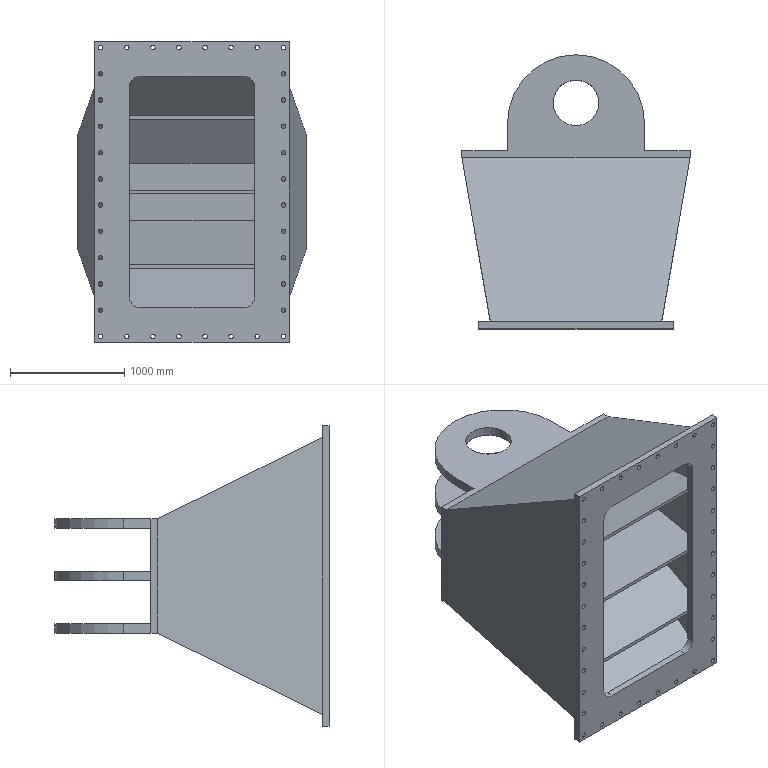Component | SolidWorks | FlexibleLegSaddleBody-1 | 1 solid | 146 faces | volume 1156094974 mm3 | cylinder 88 | plane 58 | commonest cylinder face diameters 40 x72 400 x6 1200 x6 200 x4